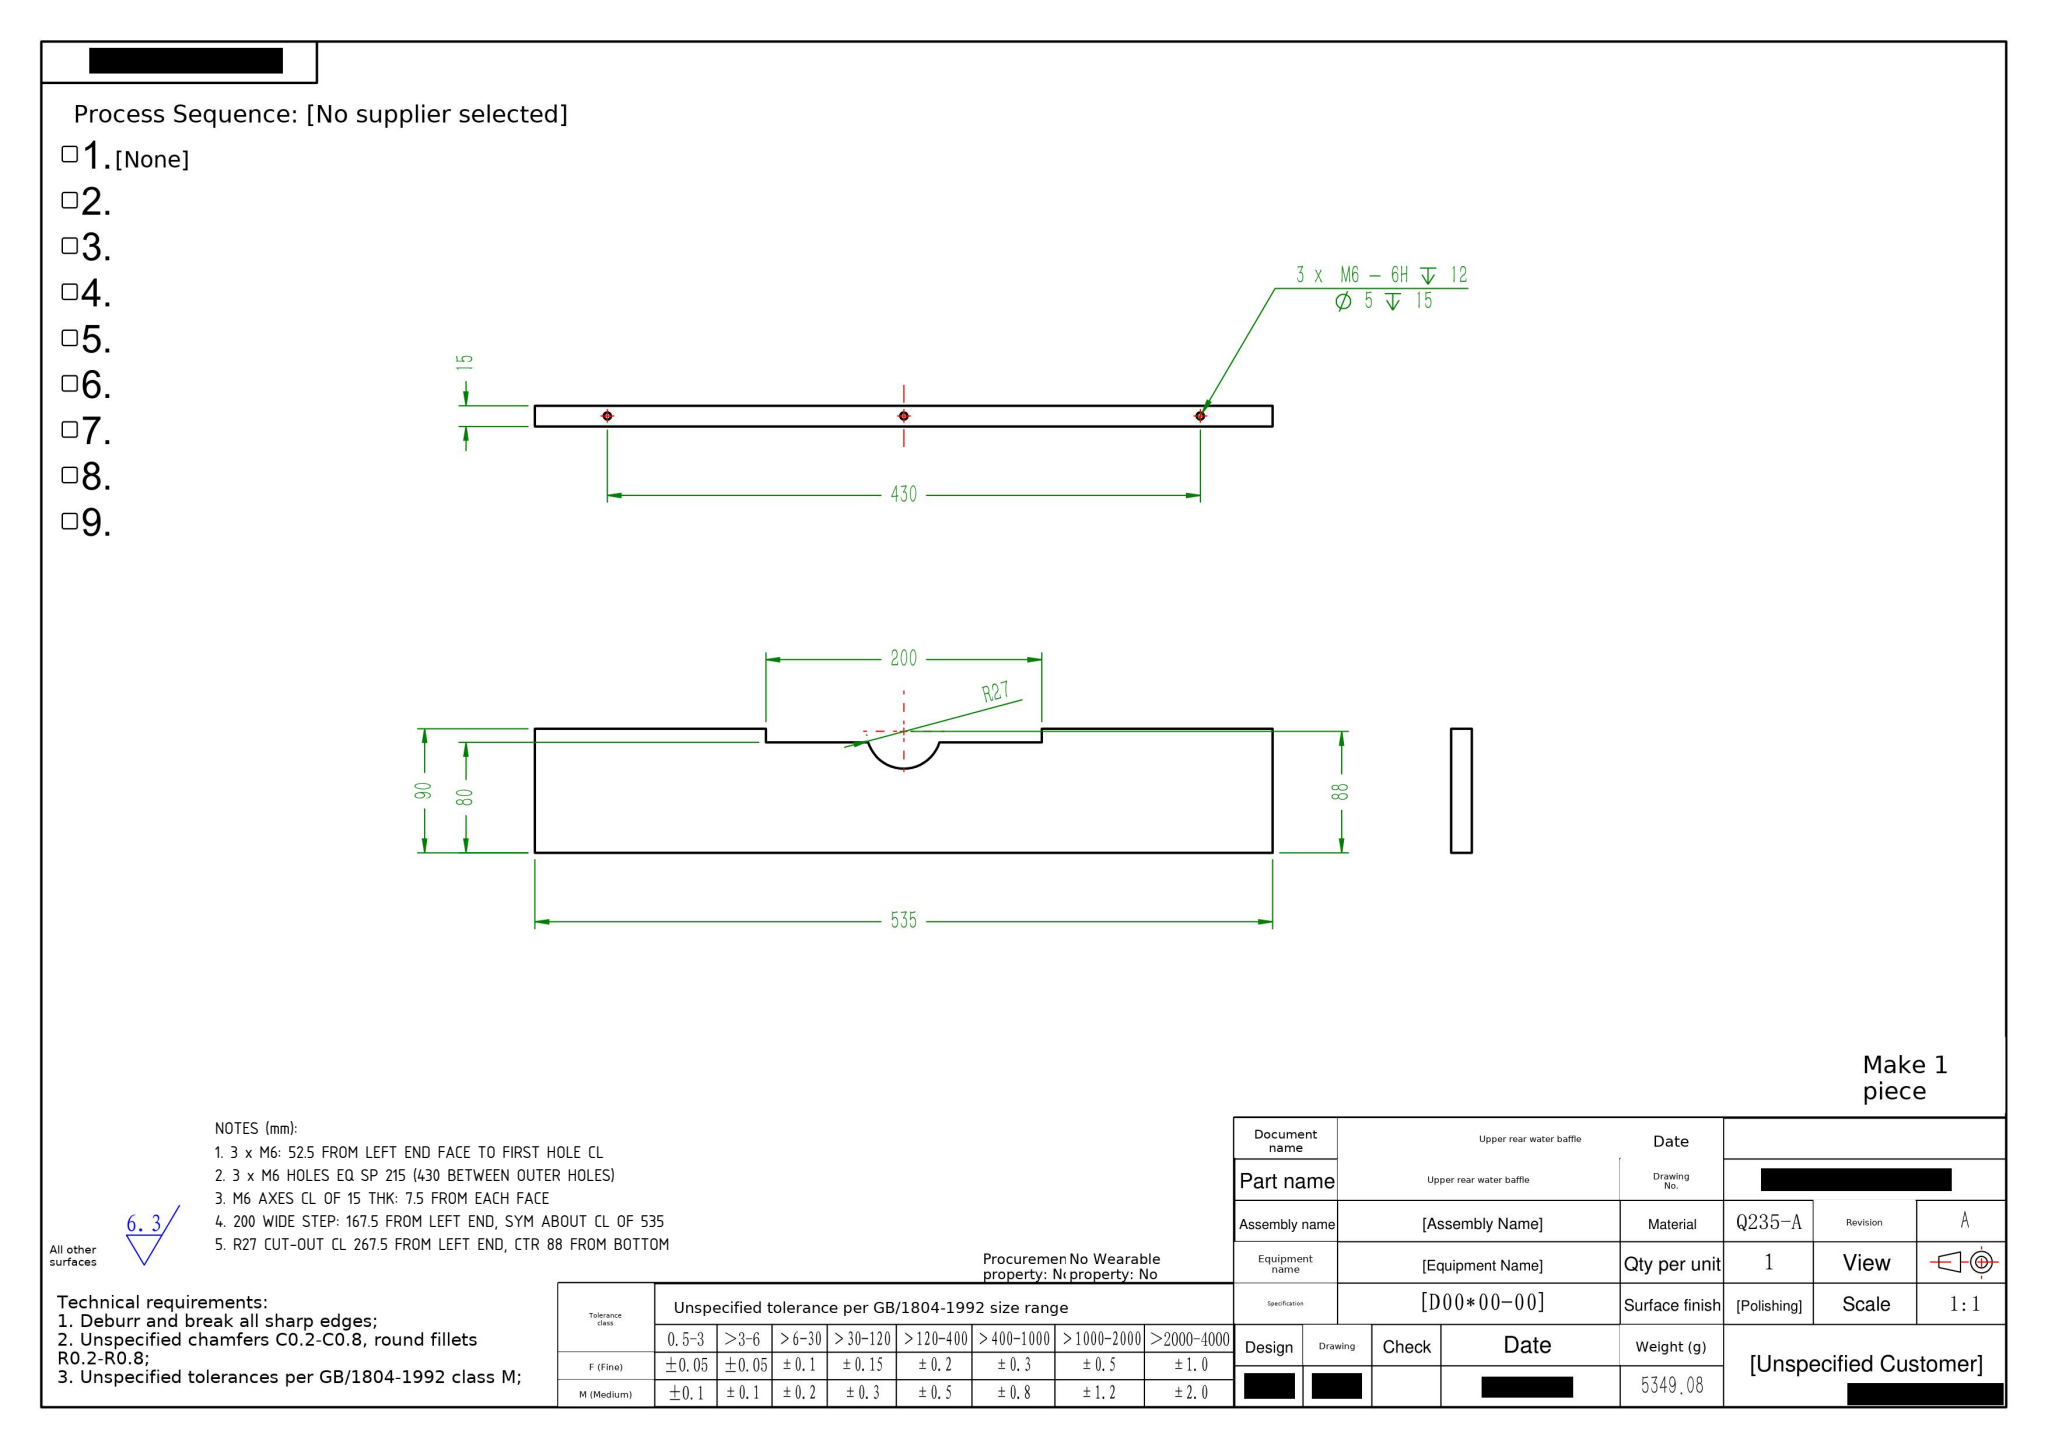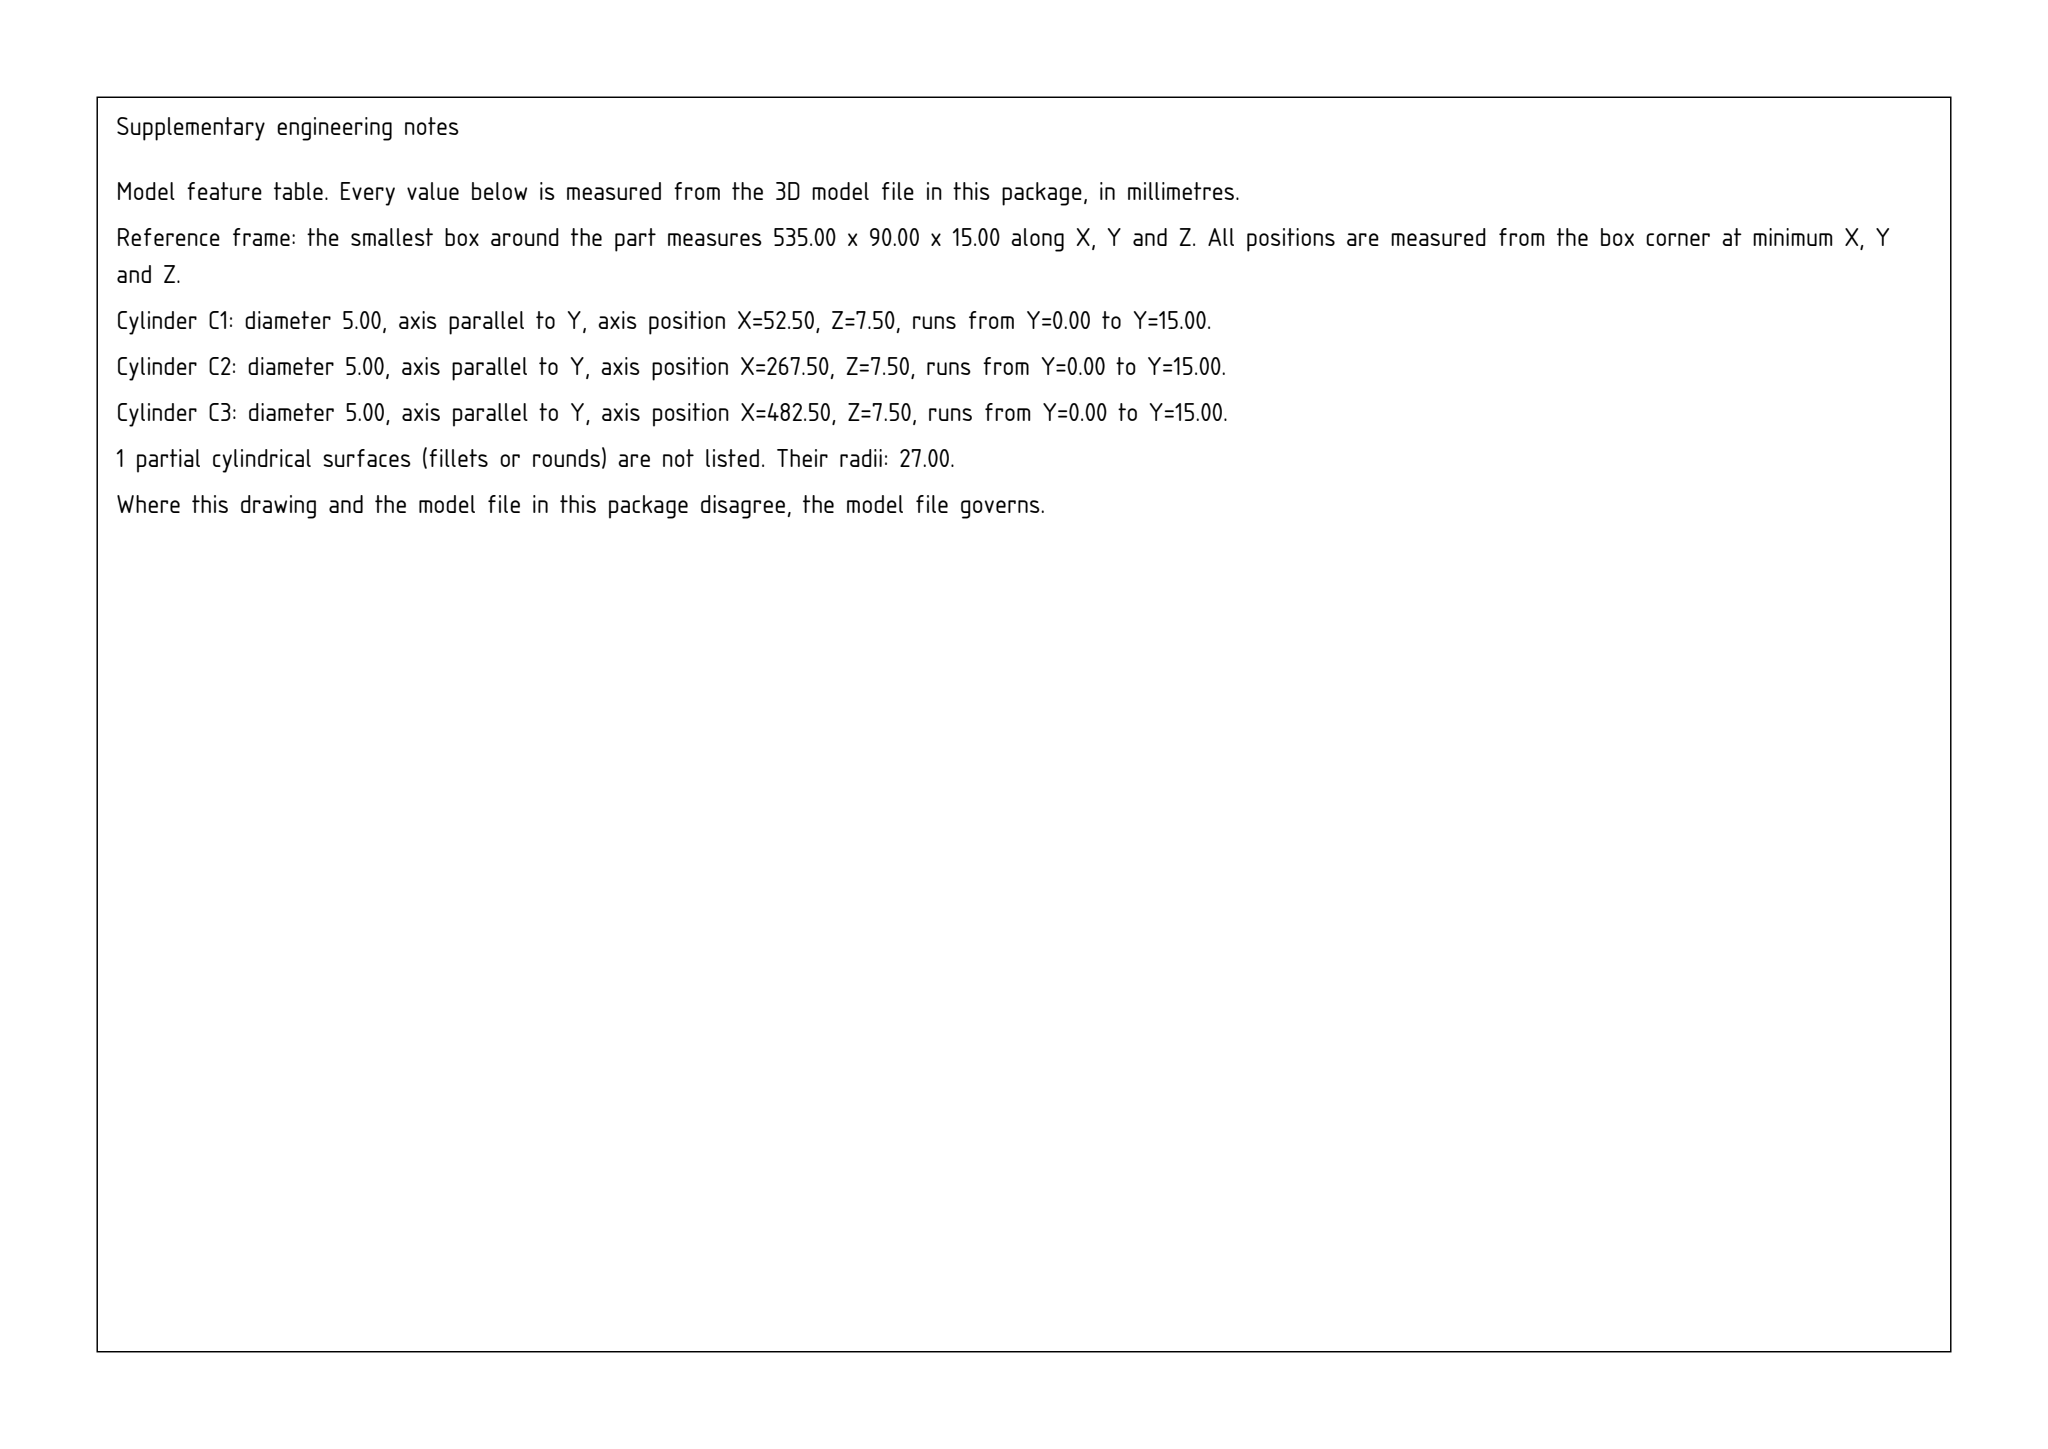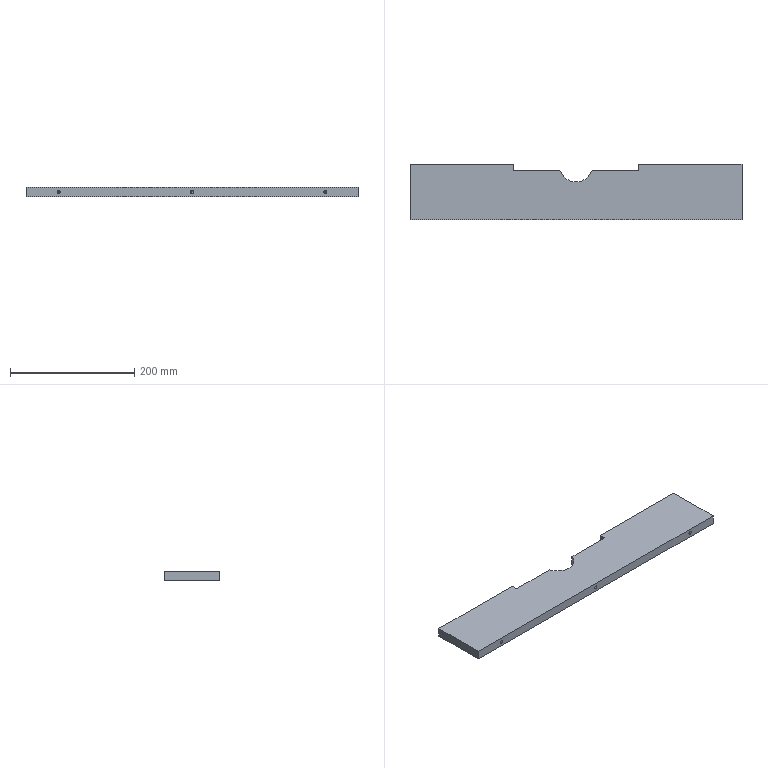Part | SolidWorks | mm | material Q235-A | 1 solid | 24 faces | box 535 x 90 x 15 mm | volume 680544 mm3 | plane 11 | cylinder 7 | cone 6 | commonest cylinder face diameters 5 x6 54 x1
Drawing notes:
3 x M6: 52.5 FROM LEFT END FACE TO FIRST HOLE CL | from the solid: Ø5 cyl axes at x=52.5, 267.5, 482.5; bbox x=535
3 x M6 HOLES EQ SP 215 (430 BETWEEN OUTER HOLES) | from the solid: hole x = 52.5 / 267.5 / 482.5 -> 215 pitch
M6 AXES CL OF 15 THK: 7.5 FROM EACH FACE | from the solid: Ø5 cyl pos z=7.5 of 15 thk
200 WIDE STEP: 167.5 FROM LEFT END, SYM ABOUT CL OF 535 | from the solid: x planes at 167.5 and 367.5; bbox x=535
R27 CUT-OUT CL 267.5 FROM LEFT END, CTR 88 FROM BOTTOM | from the solid: Ø54 cyl axis at x=267.5, y=88; bbox y=90
build123d program:
from build123d import *

# Parameters (mm, degrees)
SKETCH1_W             = 535
SKETCH1_H             = 15
BOSS_EXTRUDE1_DEPTH   = 90
M6_TAPPED_HOLE1_D     = 5
M6_TAPPED_HOLE1_DEPTH = 15
M6_TAPPED_HOLE1_TIP   = 1.502
SKETCH5_R             = 27
CUT_EXTRUDE2_DEPTH    = 283.633
SKETCH6_W             = 200
SKETCH6_H             = 16
CUT_EXTRUDE3_DEPTH    = 283.633


with BuildPart() as part:
    # Sketch1 → Boss-Extrude1 (new body)
    with BuildSketch(Plane(origin=(0, 0, 0), x_dir=(1, 0, 0), z_dir=(0, 1, 0))):
        Rectangle(SKETCH1_W, SKETCH1_H)
    extrude(amount=BOSS_EXTRUDE1_DEPTH)

    # M6 Tapped Hole1
    with Locations(Plane(origin=(0, 0, 0), x_dir=(-1, 0, 0), z_dir=(0, -1, 0))):
        with Locations((0, 0), (-215, 0), (215, 0)):
            Hole(M6_TAPPED_HOLE1_D / 2, depth=M6_TAPPED_HOLE1_DEPTH)
            with Locations((0, 0, -(M6_TAPPED_HOLE1_DEPTH + M6_TAPPED_HOLE1_TIP / 2))):  # 118° drill point
                Cone(0, M6_TAPPED_HOLE1_D / 2, M6_TAPPED_HOLE1_TIP, mode=Mode.SUBTRACT)

    # Sketch5 → Cut-Extrude2 (cut, through all)
    with BuildSketch(Plane(origin=(0, 0, -7.5), x_dir=(-1, 0, 0), z_dir=(0, 0, -1))):
        with Locations((0, 88)):
            Circle(SKETCH5_R)
    extrude(amount=-CUT_EXTRUDE2_DEPTH, mode=Mode.SUBTRACT)

    # Sketch6 → Cut-Extrude3 (cut, through all)
    with BuildSketch(Plane.XY.offset(7.5)):
        with Locations((0, 88)):
            Rectangle(SKETCH6_W, SKETCH6_H)
    extrude(amount=-CUT_EXTRUDE3_DEPTH, mode=Mode.SUBTRACT)


solid = part.part
STEP:
#1=CARTESIAN_POINT('',(0.,15.,2.5));
#2=VERTEX_POINT('',#1);
#3=CARTESIAN_POINT('',(0.,15.,-2.5));
#4=VERTEX_POINT('',#3);
#5=CARTESIAN_POINT('',(0.,15.,0.));
#6=DIRECTION('',(0.,-1.,0.));
#7=DIRECTION('',(0.,0.,-1.));
#8=AXIS2_PLACEMENT_3D('',#5,#6,#7);
#9=CIRCLE('',#8,2.5);
#10=EDGE_CURVE('',#2,#4,#9,.T.);
#11=ORIENTED_EDGE('',*,*,#10,.F.);
#12=CARTESIAN_POINT('',(0.,-0.,2.5));
#13=VERTEX_POINT('',#12);
#14=CARTESIAN_POINT('',(0.,0.,2.5));
#15=DIRECTION('',(0.,-1.,0.));
#16=VECTOR('',#15,1000.);
#17=LINE('',#14,#16);
#18=EDGE_CURVE('',#2,#13,#17,.T.);
#19=ORIENTED_EDGE('',*,*,#18,.T.);
#20=CARTESIAN_POINT('',(0.,-0.,-2.5));
#21=VERTEX_POINT('',#20);
#22=CARTESIAN_POINT('',(0.,-0.,0.));
#23=DIRECTION('',(0.,-1.,0.));
#24=DIRECTION('',(0.,0.,-1.));
#25=AXIS2_PLACEMENT_3D('',#22,#23,#24);
#26=CIRCLE('',#25,2.5);
#27=EDGE_CURVE('',#13,#21,#26,.T.);
#28=ORIENTED_EDGE('',*,*,#27,.T.);
#29=CARTESIAN_POINT('',(0.,0.,-2.5));
#30=DIRECTION('',(0.,-1.,0.));
#31=VECTOR('',#30,1000.);
#32=LINE('',#29,#31);
#33=EDGE_CURVE('',#4,#21,#32,.T.);
#34=ORIENTED_EDGE('',*,*,#33,.F.);
#35=EDGE_LOOP('',(#11,#19,#28,#34));
#36=FACE_OUTER_BOUND('',#35,.T.);
#37=CARTESIAN_POINT('',(0.,0.,0.));
#38=DIRECTION('',(0.,-1.,0.));
#39=DIRECTION('',(0.,0.,-1.));
#40=AXIS2_PLACEMENT_3D('',#37,#38,#39);
#41=CYLINDRICAL_SURFACE('',#40,2.5);
#42=ADVANCED_FACE('',(#36),#41,.F.);
#43=CARTESIAN_POINT('',(-0.,16.502,0.));
#44=VERTEX_POINT('',#43);
#45=CARTESIAN_POINT('',(0.,15.,-2.5));
#46=DIRECTION('',(0.,-0.515,-0.8572));
#47=VECTOR('',#46,1000.);
#48=LINE('',#45,#47);
#49=EDGE_CURVE('',#44,#4,#48,.T.);
#50=ORIENTED_EDGE('',*,*,#49,.F.);
#51=CARTESIAN_POINT('',(0.,15.,2.5));
#52=DIRECTION('',(0.,-0.515,0.8572));
#53=VECTOR('',#52,1000.);
#54=LINE('',#51,#53);
#55=EDGE_CURVE('',#44,#2,#54,.T.);
#56=ORIENTED_EDGE('',*,*,#55,.T.);
#57=ORIENTED_EDGE('',*,*,#10,.T.);
#58=EDGE_LOOP('',(#50,#56,#57));
#59=FACE_OUTER_BOUND('',#58,.T.);
#60=CARTESIAN_POINT('',(0.,15.,0.));
#61=DIRECTION('',(0.,-1.,0.));
#62=DIRECTION('',(0.,0.,-1.));
#63=AXIS2_PLACEMENT_3D('',#60,#61,#62);
#64=CONICAL_SURFACE('',#63,2.5,1.03);
#65=ADVANCED_FACE('',(#59),#64,.F.);
#66=CARTESIAN_POINT('',(215.,15.,2.5));
#67=VERTEX_POINT('',#66);
#68=CARTESIAN_POINT('',(215.,15.,-2.5));
#69=VERTEX_POINT('',#68);
#70=CARTESIAN_POINT('',(215.,15.,0.));
#71=DIRECTION('',(0.,-1.,0.));
#72=DIRECTION('',(0.,0.,-1.));
#73=AXIS2_PLACEMENT_3D('',#70,#71,#72);
#74=CIRCLE('',#73,2.5);
#75=EDGE_CURVE('',#67,#69,#74,.T.);
#76=ORIENTED_EDGE('',*,*,#75,.F.);
#77=CARTESIAN_POINT('',(215.,-0.,2.5));
#78=VERTEX_POINT('',#77);
#79=CARTESIAN_POINT('',(215.,0.,2.5));
#80=DIRECTION('',(0.,-1.,0.));
#81=VECTOR('',#80,1000.);
#82=LINE('',#79,#81);
#83=EDGE_CURVE('',#67,#78,#82,.T.);
#84=ORIENTED_EDGE('',*,*,#83,.T.);
#85=CARTESIAN_POINT('',(215.,-0.,-2.5));
#86=VERTEX_POINT('',#85);
#87=CARTESIAN_POINT('',(215.,-0.,0.));
#88=DIRECTION('',(0.,-1.,0.));
#89=DIRECTION('',(0.,0.,-1.));
#90=AXIS2_PLACEMENT_3D('',#87,#88,#89);
#91=CIRCLE('',#90,2.5);
#92=EDGE_CURVE('',#78,#86,#91,.T.);
#93=ORIENTED_EDGE('',*,*,#92,.T.);
#94=CARTESIAN_POINT('',(215.,0.,-2.5));
#95=DIRECTION('',(0.,-1.,0.));
#96=VECTOR('',#95,1000.);
#97=LINE('',#94,#96);
#98=EDGE_CURVE('',#69,#86,#97,.T.);
#99=ORIENTED_EDGE('',*,*,#98,.F.);
#100=EDGE_LOOP('',(#76,#84,#93,#99));
#101=FACE_OUTER_BOUND('',#100,.T.);
#102=CARTESIAN_POINT('',(215.,0.,0.));
#103=DIRECTION('',(0.,-1.,0.));
#104=DIRECTION('',(0.,0.,-1.));
#105=AXIS2_PLACEMENT_3D('',#102,#103,#104);
#106=CYLINDRICAL_SURFACE('',#105,2.5);
#107=ADVANCED_FACE('',(#101),#106,.F.);
#108=CARTESIAN_POINT('',(215.,16.502,0.));
#109=VERTEX_POINT('',#108);
#110=CARTESIAN_POINT('',(215.,15.,-2.5));
#111=DIRECTION('',(0.,-0.515,-0.8572));
#112=VECTOR('',#111,1000.);
#113=LINE('',#110,#112);
#114=EDGE_CURVE('',#109,#69,#113,.T.);
#115=ORIENTED_EDGE('',*,*,#114,.F.);
#116=CARTESIAN_POINT('',(215.,15.,2.5));
#117=DIRECTION('',(0.,-0.515,0.8572));
#118=VECTOR('',#117,1000.);
#119=LINE('',#116,#118);
#120=EDGE_CURVE('',#109,#67,#119,.T.);
#121=ORIENTED_EDGE('',*,*,#120,.T.);
#122=ORIENTED_EDGE('',*,*,#75,.T.);
#123=EDGE_LOOP('',(#115,#121,#122));
#124=FACE_OUTER_BOUND('',#123,.T.);
#125=CARTESIAN_POINT('',(215.,15.,0.));
#126=DIRECTION('',(0.,-1.,0.));
#127=DIRECTION('',(0.,0.,-1.));
#128=AXIS2_PLACEMENT_3D('',#125,#126,#127);
#129=CONICAL_SURFACE('',#128,2.5,1.03);
#130=ADVANCED_FACE('',(#124),#129,.F.);
#131=CARTESIAN_POINT('',(-215.,15.,2.5));
#132=VERTEX_POINT('',#131);
#133=CARTESIAN_POINT('',(-215.,15.,-2.5));
#134=VERTEX_POINT('',#133);
#135=CARTESIAN_POINT('',(-215.,15.,0.));
#136=DIRECTION('',(0.,-1.,0.));
#137=DIRECTION('',(0.,0.,-1.));
#138=AXIS2_PLACEMENT_3D('',#135,#136,#137);
#139=CIRCLE('',#138,2.5);
#140=EDGE_CURVE('',#132,#134,#139,.T.);
#141=ORIENTED_EDGE('',*,*,#140,.F.);
#142=CARTESIAN_POINT('',(-215.,-0.,2.5));
#143=VERTEX_POINT('',#142);
#144=CARTESIAN_POINT('',(-215.,0.,2.5));
#145=DIRECTION('',(0.,-1.,0.));
#146=VECTOR('',#145,1000.);
#147=LINE('',#144,#146);
#148=EDGE_CURVE('',#132,#143,#147,.T.);
#149=ORIENTED_EDGE('',*,*,#148,.T.);
#150=CARTESIAN_POINT('',(-215.,-0.,-2.5));
#151=VERTEX_POINT('',#150);
#152=CARTESIAN_POINT('',(-215.,-0.,0.));
#153=DIRECTION('',(0.,-1.,0.));
#154=DIRECTION('',(0.,0.,-1.));
#155=AXIS2_PLACEMENT_3D('',#152,#153,#154);
#156=CIRCLE('',#155,2.5);
#157=EDGE_CURVE('',#143,#151,#156,.T.);
#158=ORIENTED_EDGE('',*,*,#157,.T.);
#159=CARTESIAN_POINT('',(-215.,0.,-2.5));
#160=DIRECTION('',(0.,-1.,0.));
#161=VECTOR('',#160,1000.);
#162=LINE('',#159,#161);
#163=EDGE_CURVE('',#134,#151,#162,.T.);
#164=ORIENTED_EDGE('',*,*,#163,.F.);
#165=EDGE_LOOP('',(#141,#149,#158,#164));
#166=FACE_OUTER_BOUND('',#165,.T.);
#167=CARTESIAN_POINT('',(-215.,0.,0.));
#168=DIRECTION('',(0.,-1.,0.));
#169=DIRECTION('',(0.,0.,-1.));
#170=AXIS2_PLACEMENT_3D('',#167,#168,#169);
#171=CYLINDRICAL_SURFACE('',#170,2.5);
#172=ADVANCED_FACE('',(#166),#171,.F.);
#173=CARTESIAN_POINT('',(-215.,16.502,0.));
#174=VERTEX_POINT('',#173);
#175=CARTESIAN_POINT('',(-215.,15.,-2.5));
#176=DIRECTION('',(0.,-0.515,-0.8572));
#177=VECTOR('',#176,1000.);
#178=LINE('',#175,#177);
#179=EDGE_CURVE('',#174,#134,#178,.T.);
#180=ORIENTED_EDGE('',*,*,#179,.F.);
#181=CARTESIAN_POINT('',(-215.,15.,2.5));
#182=DIRECTION('',(0.,-0.515,0.8572));
#183=VECTOR('',#182,1000.);
#184=LINE('',#181,#183);
#185=EDGE_CURVE('',#174,#132,#184,.T.);
#186=ORIENTED_EDGE('',*,*,#185,.T.);
#187=ORIENTED_EDGE('',*,*,#140,.T.);
#188=EDGE_LOOP('',(#180,#186,#187));
#189=FACE_OUTER_BOUND('',#188,.T.);
#190=CARTESIAN_POINT('',(-215.,15.,0.));
#191=DIRECTION('',(0.,-1.,0.));
#192=DIRECTION('',(0.,0.,-1.));
#193=AXIS2_PLACEMENT_3D('',#190,#191,#192);
#194=CONICAL_SURFACE('',#193,2.5,1.03);
#195=ADVANCED_FACE('',(#189),#194,.F.);
#196=CARTESIAN_POINT('',(-267.5,90.,7.5));
#197=VERTEX_POINT('',#196);
#198=CARTESIAN_POINT('',(-100.,90.,7.5));
#199=VERTEX_POINT('',#198);
#200=CARTESIAN_POINT('',(267.5,90.,7.5));
#201=DIRECTION('',(1.,0.,0.));
#202=VECTOR('',#201,1000.);
#203=LINE('',#200,#202);
#204=EDGE_CURVE('',#197,#199,#203,.T.);
#205=ORIENTED_EDGE('',*,*,#204,.T.);
#206=CARTESIAN_POINT('',(-100.,90.,-7.5));
#207=VERTEX_POINT('',#206);
#208=CARTESIAN_POINT('',(-100.,90.,0.));
#209=DIRECTION('',(0.,0.,-1.));
#210=VECTOR('',#209,1000.);
#211=LINE('',#208,#210);
#212=EDGE_CURVE('',#199,#207,#211,.T.);
#213=ORIENTED_EDGE('',*,*,#212,.T.);
#214=CARTESIAN_POINT('',(-267.5,90.,-7.5));
#215=VERTEX_POINT('',#214);
#216=CARTESIAN_POINT('',(267.5,90.,-7.5));
#217=DIRECTION('',(-1.,0.,0.));
#218=VECTOR('',#217,1000.);
#219=LINE('',#216,#218);
#220=EDGE_CURVE('',#207,#215,#219,.T.);
#221=ORIENTED_EDGE('',*,*,#220,.T.);
#222=CARTESIAN_POINT('',(-267.5,90.,-7.5));
#223=DIRECTION('',(0.,0.,1.));
#224=VECTOR('',#223,1000.);
#225=LINE('',#222,#224);
#226=EDGE_CURVE('',#215,#197,#225,.T.);
#227=ORIENTED_EDGE('',*,*,#226,.T.);
#228=EDGE_LOOP('',(#205,#213,#221,#227));
#229=FACE_OUTER_BOUND('',#228,.T.);
#230=CARTESIAN_POINT('',(0.,90.,0.));
#231=DIRECTION('',(0.,-1.,0.));
#232=DIRECTION('',(0.,0.,-1.));
#233=AXIS2_PLACEMENT_3D('',#230,#231,#232);
#234=PLANE('',#233);
#235=ADVANCED_FACE('',(#229),#234,.F.);
#236=CARTESIAN_POINT('',(-267.5,0.,-7.5));
#237=VERTEX_POINT('',#236);
#238=CARTESIAN_POINT('',(-267.5,0.,7.5));
#239=VERTEX_POINT('',#238);
#240=CARTESIAN_POINT('',(-267.5,0.,-7.5));
#241=DIRECTION('',(0.,0.,1.));
#242=VECTOR('',#241,1000.);
#243=LINE('',#240,#242);
#244=EDGE_CURVE('',#237,#239,#243,.T.);
#245=ORIENTED_EDGE('',*,*,#244,.T.);
#246=CARTESIAN_POINT('',(-267.5,90.,7.5));
#247=DIRECTION('',(0.,-1.,0.));
#248=VECTOR('',#247,1000.);
#249=LINE('',#246,#248);
#250=EDGE_CURVE('',#197,#239,#249,.T.);
#251=ORIENTED_EDGE('',*,*,#250,.F.);
#252=ORIENTED_EDGE('',*,*,#226,.F.);
#253=CARTESIAN_POINT('',(-267.5,90.,-7.5));
#254=DIRECTION('',(0.,-1.,0.));
#255=VECTOR('',#254,1000.);
#256=LINE('',#253,#255);
#257=EDGE_CURVE('',#215,#237,#256,.T.);
#258=ORIENTED_EDGE('',*,*,#257,.T.);
#259=EDGE_LOOP('',(#245,#251,#252,#258));
#260=FACE_OUTER_BOUND('',#259,.T.);
#261=CARTESIAN_POINT('',(-267.5,90.,-7.5));
#262=DIRECTION('',(1.,0.,0.));
#263=DIRECTION('',(0.,0.,-1.));
#264=AXIS2_PLACEMENT_3D('',#261,#262,#263);
#265=PLANE('',#264);
#266=ADVANCED_FACE('',(#260),#265,.F.);
#267=CARTESIAN_POINT('',(100.,90.,7.5));
#268=VERTEX_POINT('',#267);
#269=CARTESIAN_POINT('',(267.5,90.,7.5));
#270=VERTEX_POINT('',#269);
#271=CARTESIAN_POINT('',(267.5,90.,7.5));
#272=DIRECTION('',(1.,0.,0.));
#273=VECTOR('',#272,1000.);
#274=LINE('',#271,#273);
#275=EDGE_CURVE('',#268,#270,#274,.T.);
#276=ORIENTED_EDGE('',*,*,#275,.F.);
#277=CARTESIAN_POINT('',(100.,80.,7.5));
#278=VERTEX_POINT('',#277);
#279=CARTESIAN_POINT('',(100.,96.,7.5));
#280=DIRECTION('',(0.,1.,0.));
#281=VECTOR('',#280,1000.);
#282=LINE('',#279,#281);
#283=EDGE_CURVE('',#278,#268,#282,.T.);
#284=ORIENTED_EDGE('',*,*,#283,.F.);
#285=CARTESIAN_POINT('',(25.788,80.,7.5));
#286=VERTEX_POINT('',#285);
#287=CARTESIAN_POINT('',(100.,80.,7.5));
#288=DIRECTION('',(1.,0.,0.));
#289=VECTOR('',#288,1000.);
#290=LINE('',#287,#289);
#291=EDGE_CURVE('',#286,#278,#290,.T.);
#292=ORIENTED_EDGE('',*,*,#291,.F.);
#293=CARTESIAN_POINT('',(-25.788,80.,7.5));
#294=VERTEX_POINT('',#293);
#295=CARTESIAN_POINT('',(0.,88.,7.5));
#296=DIRECTION('',(0.,0.,-1.));
#297=DIRECTION('',(-1.,0.,0.));
#298=AXIS2_PLACEMENT_3D('',#295,#296,#297);
#299=CIRCLE('',#298,27.);
#300=EDGE_CURVE('',#286,#294,#299,.T.);
#301=ORIENTED_EDGE('',*,*,#300,.T.);
#302=CARTESIAN_POINT('',(-100.,80.,7.5));
#303=VERTEX_POINT('',#302);
#304=CARTESIAN_POINT('',(100.,80.,7.5));
#305=DIRECTION('',(1.,0.,0.));
#306=VECTOR('',#305,1000.);
#307=LINE('',#304,#306);
#308=EDGE_CURVE('',#303,#294,#307,.T.);
#309=ORIENTED_EDGE('',*,*,#308,.F.);
#310=CARTESIAN_POINT('',(-100.,96.,7.5));
#311=DIRECTION('',(0.,-1.,0.));
#312=VECTOR('',#311,1000.);
#313=LINE('',#310,#312);
#314=EDGE_CURVE('',#199,#303,#313,.T.);
#315=ORIENTED_EDGE('',*,*,#314,.F.);
#316=ORIENTED_EDGE('',*,*,#204,.F.);
#317=ORIENTED_EDGE('',*,*,#250,.T.);
#318=CARTESIAN_POINT('',(267.5,0.,7.5));
#319=VERTEX_POINT('',#318);
#320=CARTESIAN_POINT('',(267.5,0.,7.5));
#321=DIRECTION('',(1.,0.,0.));
#322=VECTOR('',#321,1000.);
#323=LINE('',#320,#322);
#324=EDGE_CURVE('',#239,#319,#323,.T.);
#325=ORIENTED_EDGE('',*,*,#324,.T.);
#326=CARTESIAN_POINT('',(267.5,90.,7.5));
#327=DIRECTION('',(0.,-1.,0.));
#328=VECTOR('',#327,1000.);
#329=LINE('',#326,#328);
#330=EDGE_CURVE('',#270,#319,#329,.T.);
#331=ORIENTED_EDGE('',*,*,#330,.F.);
#332=EDGE_LOOP('',(#276,#284,#292,#301,#309,#315,#316,#317,#325,#331));
#333=FACE_OUTER_BOUND('',#332,.T.);
#334=CARTESIAN_POINT('',(267.5,90.,7.5));
#335=DIRECTION('',(0.,0.,-1.));
#336=DIRECTION('',(-1.,0.,0.));
#337=AXIS2_PLACEMENT_3D('',#334,#335,#336);
#338=PLANE('',#337);
#339=ADVANCED_FACE('',(#333),#338,.F.);
#340=CARTESIAN_POINT('',(267.5,0.,-7.5));
#341=VERTEX_POINT('',#340);
#342=CARTESIAN_POINT('',(267.5,0.,-7.5));
#343=DIRECTION('',(0.,0.,-1.));
#344=VECTOR('',#343,1000.);
#345=LINE('',#342,#344);
#346=EDGE_CURVE('',#319,#341,#345,.T.);
#347=ORIENTED_EDGE('',*,*,#346,.T.);
#348=CARTESIAN_POINT('',(267.5,90.,-7.5));
#349=VERTEX_POINT('',#348);
#350=CARTESIAN_POINT('',(267.5,90.,-7.5));
#351=DIRECTION('',(0.,-1.,0.));
#352=VECTOR('',#351,1000.);
#353=LINE('',#350,#352);
#354=EDGE_CURVE('',#349,#341,#353,.T.);
#355=ORIENTED_EDGE('',*,*,#354,.F.);
#356=CARTESIAN_POINT('',(267.5,90.,-7.5));
#357=DIRECTION('',(0.,0.,-1.));
#358=VECTOR('',#357,1000.);
#359=LINE('',#356,#358);
#360=EDGE_CURVE('',#270,#349,#359,.T.);
#361=ORIENTED_EDGE('',*,*,#360,.F.);
#362=ORIENTED_EDGE('',*,*,#330,.T.);
#363=EDGE_LOOP('',(#347,#355,#361,#362));
#364=FACE_OUTER_BOUND('',#363,.T.);
#365=CARTESIAN_POINT('',(267.5,90.,-7.5));
#366=DIRECTION('',(-1.,0.,0.));
#367=DIRECTION('',(0.,0.,1.));
#368=AXIS2_PLACEMENT_3D('',#365,#366,#367);
#369=PLANE('',#368);
#370=ADVANCED_FACE('',(#364),#369,.F.);
#371=ORIENTED_EDGE('',*,*,#220,.F.);
#372=CARTESIAN_POINT('',(-100.,80.,-7.5));
#373=VERTEX_POINT('',#372);
#374=CARTESIAN_POINT('',(-100.,96.,-7.5));
#375=DIRECTION('',(0.,-1.,0.));
#376=VECTOR('',#375,1000.);
#377=LINE('',#374,#376);
#378=EDGE_CURVE('',#207,#373,#377,.T.);
#379=ORIENTED_EDGE('',*,*,#378,.T.);
#380=CARTESIAN_POINT('',(-25.788,80.,-7.5));
#381=VERTEX_POINT('',#380);
#382=CARTESIAN_POINT('',(100.,80.,-7.5));
#383=DIRECTION('',(1.,0.,0.));
#384=VECTOR('',#383,1000.);
#385=LINE('',#382,#384);
#386=EDGE_CURVE('',#373,#381,#385,.T.);
#387=ORIENTED_EDGE('',*,*,#386,.T.);
#388=CARTESIAN_POINT('',(25.788,80.,-7.5));
#389=VERTEX_POINT('',#388);
#390=CARTESIAN_POINT('',(0.,88.,-7.5));
#391=DIRECTION('',(0.,0.,-1.));
#392=DIRECTION('',(-1.,0.,0.));
#393=AXIS2_PLACEMENT_3D('',#390,#391,#392);
#394=CIRCLE('',#393,27.);
#395=EDGE_CURVE('',#389,#381,#394,.T.);
#396=ORIENTED_EDGE('',*,*,#395,.F.);
#397=CARTESIAN_POINT('',(100.,80.,-7.5));
#398=VERTEX_POINT('',#397);
#399=CARTESIAN_POINT('',(100.,80.,-7.5));
#400=DIRECTION('',(1.,0.,0.));
#401=VECTOR('',#400,1000.);
#402=LINE('',#399,#401);
#403=EDGE_CURVE('',#389,#398,#402,.T.);
#404=ORIENTED_EDGE('',*,*,#403,.T.);
#405=CARTESIAN_POINT('',(100.,90.,-7.5));
#406=VERTEX_POINT('',#405);
#407=CARTESIAN_POINT('',(100.,96.,-7.5));
#408=DIRECTION('',(0.,1.,0.));
#409=VECTOR('',#408,1000.);
#410=LINE('',#407,#409);
#411=EDGE_CURVE('',#398,#406,#410,.T.);
#412=ORIENTED_EDGE('',*,*,#411,.T.);
#413=CARTESIAN_POINT('',(267.5,90.,-7.5));
#414=DIRECTION('',(-1.,0.,0.));
#415=VECTOR('',#414,1000.);
#416=LINE('',#413,#415);
#417=EDGE_CURVE('',#349,#406,#416,.T.);
#418=ORIENTED_EDGE('',*,*,#417,.F.);
#419=ORIENTED_EDGE('',*,*,#354,.T.);
#420=CARTESIAN_POINT('',(267.5,0.,-7.5));
#421=DIRECTION('',(-1.,0.,0.));
#422=VECTOR('',#421,1000.);
#423=LINE('',#420,#422);
#424=EDGE_CURVE('',#341,#237,#423,.T.);
#425=ORIENTED_EDGE('',*,*,#424,.T.);
#426=ORIENTED_EDGE('',*,*,#257,.F.);
#427=EDGE_LOOP('',(#371,#379,#387,#396,#404,#412,#418,#419,#425,#426));
#428=FACE_OUTER_BOUND('',#427,.T.);
#429=CARTESIAN_POINT('',(267.5,90.,-7.5));
#430=DIRECTION('',(0.,0.,1.));
#431=DIRECTION('',(1.,0.,0.));
#432=AXIS2_PLACEMENT_3D('',#429,#430,#431);
#433=PLANE('',#432);
#434=ADVANCED_FACE('',(#428),#433,.F.);
#435=ORIENTED_EDGE('',*,*,#417,.T.);
#436=CARTESIAN_POINT('',(100.,90.,0.));
#437=DIRECTION('',(0.,0.,1.));
#438=VECTOR('',#437,1000.);
#439=LINE('',#436,#438);
#440=EDGE_CURVE('',#406,#268,#439,.T.);
#441=ORIENTED_EDGE('',*,*,#440,.T.);
#442=ORIENTED_EDGE('',*,*,#275,.T.);
#443=ORIENTED_EDGE('',*,*,#360,.T.);
#444=EDGE_LOOP('',(#435,#441,#442,#443));
#445=FACE_OUTER_BOUND('',#444,.T.);
#446=CARTESIAN_POINT('',(0.,90.,0.));
#447=DIRECTION('',(0.,-1.,0.));
#448=DIRECTION('',(0.,0.,-1.));
#449=AXIS2_PLACEMENT_3D('',#446,#447,#448);
#450=PLANE('',#449);
#451=ADVANCED_FACE('',(#445),#450,.F.);
#452=CARTESIAN_POINT('',(0.,-0.,0.));
#453=DIRECTION('',(0.,-1.,0.));
#454=DIRECTION('',(0.,0.,-1.));
#455=AXIS2_PLACEMENT_3D('',#452,#453,#454);
#456=CIRCLE('',#455,2.5);
#457=EDGE_CURVE('',#21,#13,#456,.T.);
#458=ORIENTED_EDGE('',*,*,#457,.F.);
#459=ORIENTED_EDGE('',*,*,#27,.F.);
#460=EDGE_LOOP('',(#458,#459));
#461=FACE_BOUND('',#460,.T.);
#462=CARTESIAN_POINT('',(215.,-0.,0.));
#463=DIRECTION('',(0.,-1.,0.));
#464=DIRECTION('',(0.,0.,-1.));
#465=AXIS2_PLACEMENT_3D('',#462,#463,#464);
#466=CIRCLE('',#465,2.5);
#467=EDGE_CURVE('',#86,#78,#466,.T.);
#468=ORIENTED_EDGE('',*,*,#467,.F.);
#469=ORIENTED_EDGE('',*,*,#92,.F.);
#470=EDGE_LOOP('',(#468,#469));
#471=FACE_BOUND('',#470,.T.);
#472=CARTESIAN_POINT('',(-215.,-0.,0.));
#473=DIRECTION('',(0.,-1.,0.));
#474=DIRECTION('',(0.,0.,-1.));
#475=AXIS2_PLACEMENT_3D('',#472,#473,#474);
#476=CIRCLE('',#475,2.5);
#477=EDGE_CURVE('',#151,#143,#476,.T.);
#478=ORIENTED_EDGE('',*,*,#477,.F.);
#479=ORIENTED_EDGE('',*,*,#157,.F.);
#480=EDGE_LOOP('',(#478,#479));
#481=FACE_BOUND('',#480,.T.);
#482=ORIENTED_EDGE('',*,*,#244,.F.);
#483=ORIENTED_EDGE('',*,*,#424,.F.);
#484=ORIENTED_EDGE('',*,*,#346,.F.);
#485=ORIENTED_EDGE('',*,*,#324,.F.);
#486=EDGE_LOOP('',(#482,#483,#484,#485));
#487=FACE_OUTER_BOUND('',#486,.T.);
#488=CARTESIAN_POINT('',(0.,0.,0.));
#489=DIRECTION('',(0.,-1.,0.));
#490=DIRECTION('',(0.,0.,-1.));
#491=AXIS2_PLACEMENT_3D('',#488,#489,#490);
#492=PLANE('',#491);
#493=ADVANCED_FACE('',(#461,#471,#481,#487),#492,.T.);
#494=ORIENTED_EDGE('',*,*,#185,.F.);
#495=ORIENTED_EDGE('',*,*,#179,.T.);
#496=CARTESIAN_POINT('',(-215.,15.,0.));
#497=DIRECTION('',(0.,-1.,0.));
#498=DIRECTION('',(0.,0.,-1.));
#499=AXIS2_PLACEMENT_3D('',#496,#497,#498);
#500=CIRCLE('',#499,2.5);
#501=EDGE_CURVE('',#134,#132,#500,.T.);
#502=ORIENTED_EDGE('',*,*,#501,.T.);
#503=EDGE_LOOP('',(#494,#495,#502));
#504=FACE_OUTER_BOUND('',#503,.T.);
#505=CARTESIAN_POINT('',(-215.,15.,0.));
#506=DIRECTION('',(0.,-1.,0.));
#507=DIRECTION('',(0.,0.,-1.));
#508=AXIS2_PLACEMENT_3D('',#505,#506,#507);
#509=CONICAL_SURFACE('',#508,2.5,1.03);
#510=ADVANCED_FACE('',(#504),#509,.F.);
#511=ORIENTED_EDGE('',*,*,#148,.F.);
#512=ORIENTED_EDGE('',*,*,#501,.F.);
#513=ORIENTED_EDGE('',*,*,#163,.T.);
#514=ORIENTED_EDGE('',*,*,#477,.T.);
#515=EDGE_LOOP('',(#511,#512,#513,#514));
#516=FACE_OUTER_BOUND('',#515,.T.);
#517=CARTESIAN_POINT('',(-215.,0.,0.));
#518=DIRECTION('',(0.,-1.,0.));
#519=DIRECTION('',(0.,0.,-1.));
#520=AXIS2_PLACEMENT_3D('',#517,#518,#519);
#521=CYLINDRICAL_SURFACE('',#520,2.5);
#522=ADVANCED_FACE('',(#516),#521,.F.);
#523=ORIENTED_EDGE('',*,*,#120,.F.);
#524=ORIENTED_EDGE('',*,*,#114,.T.);
#525=CARTESIAN_POINT('',(215.,15.,0.));
#526=DIRECTION('',(0.,-1.,0.));
#527=DIRECTION('',(0.,0.,-1.));
#528=AXIS2_PLACEMENT_3D('',#525,#526,#527);
#529=CIRCLE('',#528,2.5);
#530=EDGE_CURVE('',#69,#67,#529,.T.);
#531=ORIENTED_EDGE('',*,*,#530,.T.);
#532=EDGE_LOOP('',(#523,#524,#531));
#533=FACE_OUTER_BOUND('',#532,.T.);
#534=CARTESIAN_POINT('',(215.,15.,0.));
#535=DIRECTION('',(0.,-1.,0.));
#536=DIRECTION('',(0.,0.,-1.));
#537=AXIS2_PLACEMENT_3D('',#534,#535,#536);
#538=CONICAL_SURFACE('',#537,2.5,1.03);
#539=ADVANCED_FACE('',(#533),#538,.F.);
#540=ORIENTED_EDGE('',*,*,#83,.F.);
#541=ORIENTED_EDGE('',*,*,#530,.F.);
#542=ORIENTED_EDGE('',*,*,#98,.T.);
#543=ORIENTED_EDGE('',*,*,#467,.T.);
#544=EDGE_LOOP('',(#540,#541,#542,#543));
#545=FACE_OUTER_BOUND('',#544,.T.);
#546=CARTESIAN_POINT('',(215.,0.,0.));
#547=DIRECTION('',(0.,-1.,0.));
#548=DIRECTION('',(0.,0.,-1.));
#549=AXIS2_PLACEMENT_3D('',#546,#547,#548);
#550=CYLINDRICAL_SURFACE('',#549,2.5);
#551=ADVANCED_FACE('',(#545),#550,.F.);
#552=ORIENTED_EDGE('',*,*,#55,.F.);
#553=ORIENTED_EDGE('',*,*,#49,.T.);
#554=CARTESIAN_POINT('',(0.,15.,0.));
#555=DIRECTION('',(0.,-1.,0.));
#556=DIRECTION('',(0.,0.,-1.));
#557=AXIS2_PLACEMENT_3D('',#554,#555,#556);
#558=CIRCLE('',#557,2.5);
#559=EDGE_CURVE('',#4,#2,#558,.T.);
#560=ORIENTED_EDGE('',*,*,#559,.T.);
#561=EDGE_LOOP('',(#552,#553,#560));
#562=FACE_OUTER_BOUND('',#561,.T.);
#563=CARTESIAN_POINT('',(0.,15.,0.));
#564=DIRECTION('',(0.,-1.,0.));
#565=DIRECTION('',(0.,0.,-1.));
#566=AXIS2_PLACEMENT_3D('',#563,#564,#565);
#567=CONICAL_SURFACE('',#566,2.5,1.03);
#568=ADVANCED_FACE('',(#562),#567,.F.);
#569=ORIENTED_EDGE('',*,*,#18,.F.);
#570=ORIENTED_EDGE('',*,*,#559,.F.);
#571=ORIENTED_EDGE('',*,*,#33,.T.);
#572=ORIENTED_EDGE('',*,*,#457,.T.);
#573=EDGE_LOOP('',(#569,#570,#571,#572));
#574=FACE_OUTER_BOUND('',#573,.T.);
#575=CARTESIAN_POINT('',(0.,0.,0.));
#576=DIRECTION('',(0.,-1.,0.));
#577=DIRECTION('',(0.,0.,-1.));
#578=AXIS2_PLACEMENT_3D('',#575,#576,#577);
#579=CYLINDRICAL_SURFACE('',#578,2.5);
#580=ADVANCED_FACE('',(#574),#579,.F.);
#581=ORIENTED_EDGE('',*,*,#395,.T.);
#582=CARTESIAN_POINT('',(-25.788,80.,7.5));
#583=DIRECTION('',(0.,0.,1.));
#584=VECTOR('',#583,1000.);
#585=LINE('',#582,#584);
#586=EDGE_CURVE('',#381,#294,#585,.T.);
#587=ORIENTED_EDGE('',*,*,#586,.T.);
#588=ORIENTED_EDGE('',*,*,#300,.F.);
#589=CARTESIAN_POINT('',(25.788,80.,7.5));
#590=DIRECTION('',(0.,0.,-1.));
#591=VECTOR('',#590,1000.);
#592=LINE('',#589,#591);
#593=EDGE_CURVE('',#286,#389,#592,.T.);
#594=ORIENTED_EDGE('',*,*,#593,.T.);
#595=EDGE_LOOP('',(#581,#587,#588,#594));
#596=FACE_OUTER_BOUND('',#595,.T.);
#597=CARTESIAN_POINT('',(0.,88.,7.5));
#598=DIRECTION('',(0.,0.,-1.));
#599=DIRECTION('',(-1.,0.,0.));
#600=AXIS2_PLACEMENT_3D('',#597,#598,#599);
#601=CYLINDRICAL_SURFACE('',#600,27.);
#602=ADVANCED_FACE('',(#596),#601,.F.);
#603=ORIENTED_EDGE('',*,*,#291,.T.);
#604=CARTESIAN_POINT('',(100.,80.,-7.5));
#605=DIRECTION('',(0.,0.,1.));
#606=VECTOR('',#605,1000.);
#607=LINE('',#604,#606);
#608=EDGE_CURVE('',#398,#278,#607,.T.);
#609=ORIENTED_EDGE('',*,*,#608,.F.);
#610=ORIENTED_EDGE('',*,*,#403,.F.);
#611=ORIENTED_EDGE('',*,*,#593,.F.);
#612=EDGE_LOOP('',(#603,#609,#610,#611));
#613=FACE_OUTER_BOUND('',#612,.T.);
#614=CARTESIAN_POINT('',(100.,80.,-7.5));
#615=DIRECTION('',(0.,-1.,0.));
#616=DIRECTION('',(1.,0.,0.));
#617=AXIS2_PLACEMENT_3D('',#614,#615,#616);
#618=PLANE('',#617);
#619=ADVANCED_FACE('',(#613),#618,.F.);
#620=ORIENTED_EDGE('',*,*,#411,.F.);
#621=ORIENTED_EDGE('',*,*,#608,.T.);
#622=ORIENTED_EDGE('',*,*,#283,.T.);
#623=ORIENTED_EDGE('',*,*,#440,.F.);
#624=EDGE_LOOP('',(#620,#621,#622,#623));
#625=FACE_OUTER_BOUND('',#624,.T.);
#626=CARTESIAN_POINT('',(100.,96.,-7.5));
#627=DIRECTION('',(1.,0.,0.));
#628=DIRECTION('',(0.,0.,-1.));
#629=AXIS2_PLACEMENT_3D('',#626,#627,#628);
#630=PLANE('',#629);
#631=ADVANCED_FACE('',(#625),#630,.F.);
#632=ORIENTED_EDGE('',*,*,#314,.T.);
#633=CARTESIAN_POINT('',(-100.,80.,-7.5));
#634=DIRECTION('',(0.,0.,1.));
#635=VECTOR('',#634,1000.);
#636=LINE('',#633,#635);
#637=EDGE_CURVE('',#373,#303,#636,.T.);
#638=ORIENTED_EDGE('',*,*,#637,.F.);
#639=ORIENTED_EDGE('',*,*,#378,.F.);
#640=ORIENTED_EDGE('',*,*,#212,.F.);
#641=EDGE_LOOP('',(#632,#638,#639,#640));
#642=FACE_OUTER_BOUND('',#641,.T.);
#643=CARTESIAN_POINT('',(-100.,96.,-7.5));
#644=DIRECTION('',(-1.,0.,0.));
#645=DIRECTION('',(0.,0.,1.));
#646=AXIS2_PLACEMENT_3D('',#643,#644,#645);
#647=PLANE('',#646);
#648=ADVANCED_FACE('',(#642),#647,.F.);
#649=ORIENTED_EDGE('',*,*,#386,.F.);
#650=ORIENTED_EDGE('',*,*,#637,.T.);
#651=ORIENTED_EDGE('',*,*,#308,.T.);
#652=ORIENTED_EDGE('',*,*,#586,.F.);
#653=EDGE_LOOP('',(#649,#650,#651,#652));
#654=FACE_OUTER_BOUND('',#653,.T.);
#655=CARTESIAN_POINT('',(100.,80.,-7.5));
#656=DIRECTION('',(0.,-1.,0.));
#657=DIRECTION('',(1.,0.,0.));
#658=AXIS2_PLACEMENT_3D('',#655,#656,#657);
#659=PLANE('',#658);
#660=ADVANCED_FACE('',(#654),#659,.F.);
#661=CLOSED_SHELL('',(#42,#65,#107,#130,#172,#195,#235,#266,#339,#370,#434,#451,#493,#510,#522,#539,#551,#568,#580,#602,#619,#631,#648,#660));
#662=MANIFOLD_SOLID_BREP('',#661);
#663=CARTESIAN_POINT('',(0.,0.,0.));
#664=DIRECTION('',(0.,0.,1.));
#665=DIRECTION('',(1.,0.,0.));
#666=AXIS2_PLACEMENT_3D('',#663,#664,#665);
#667=(LENGTH_UNIT()NAMED_UNIT(*)SI_UNIT(.MILLI.,.METRE.));
#668=UNCERTAINTY_MEASURE_WITH_UNIT(LENGTH_MEASURE(0.00001),#667,'','');
#669=(NAMED_UNIT(*)PLANE_ANGLE_UNIT()SI_UNIT($,.RADIAN.));
#670=(NAMED_UNIT(*)SI_UNIT($,.STERADIAN.)SOLID_ANGLE_UNIT());
#671=(GEOMETRIC_REPRESENTATION_CONTEXT(3)GLOBAL_UNCERTAINTY_ASSIGNED_CONTEXT((#668))GLOBAL_UNIT_ASSIGNED_CONTEXT((#667,#669,#670))REPRESENTATION_CONTEXT('',''));
#672=ADVANCED_BREP_SHAPE_REPRESENTATION('',(#662,#666),#671);